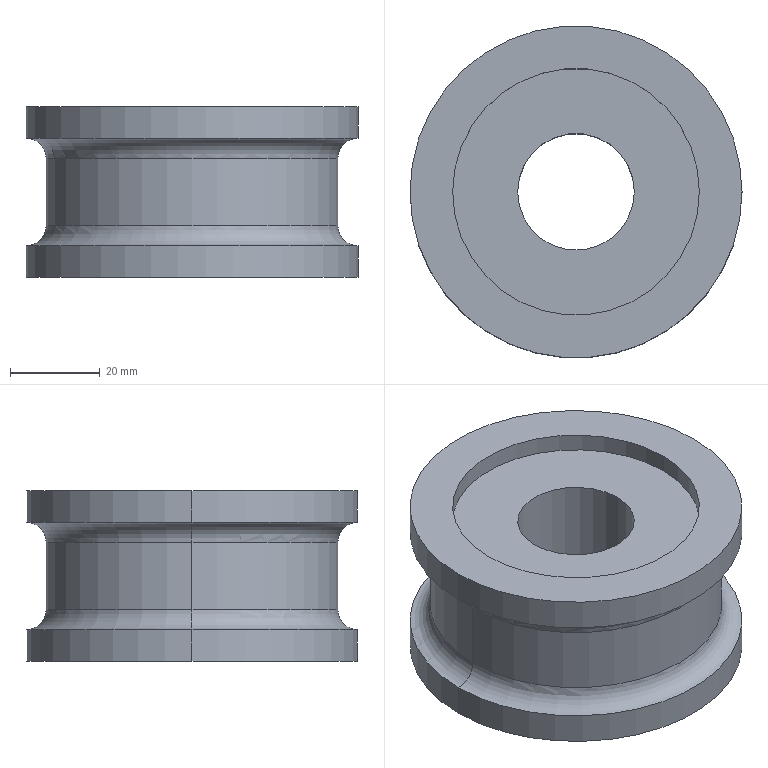Component | SolidWorks | 12AFlatGrooveSmallWheel-MillingAxis-1_12AFlatSlotSmallStraighteningWheel-1 | 1 solid | 20 faces | box 74 x 74 x 38 mm | volume 106746 mm3 | cylinder 12 | torus 4 | plane 4 | commonest cylinder face diameters 55 x4 74 x4 26 x2 65 x2 | material GCr15
build123d program:
from build123d import *


with BuildPart() as part:
    # Sketch1 → Revolve1 (revolve)
    with BuildSketch(Plane.XY, mode=Mode.PRIVATE) as revolve1_sk:
        with BuildLine():
            Line((0, 27.5), (0, 37))
            Line((0, 37), (7, 37))
            ThreePointArc((7, 37), (8.318, 33.818), (11.5, 32.5))
            Line((11.5, 32.5), (26.5, 32.5))
            ThreePointArc((26.5, 32.5), (29.682, 33.818), (31, 37))
            Line((31, 37), (38, 37))
            Line((38, 37), (38, 27.5))
            Line((38, 27.5), (34, 27.5))
            Line((34, 27.5), (34, 13))
            Line((34, 13), (4, 13))
            Line((4, 13), (4, 27.5))
            Line((4, 27.5), (0, 27.5))
        make_face()
    revolve(revolve1_sk.sketch.rotate(Axis((0, 0, 0), (1, 0, 0)), 90), axis=Axis((0, 0, 0), (1, 0, 0)))


solid = part.part

# Placed as in the assembly
solid = solid.moved(Location((-170.402, 66.538, 55.75), (0, 90, 0)))
STEP:
#1=CARTESIAN_POINT('',(-7.221,2.62,0.8563));
#2=VERTEX_POINT('',#1);
#3=CARTESIAN_POINT('',(-6.197,2.62,0.8563));
#4=VERTEX_POINT('',#3);
#5=CARTESIAN_POINT('',(-6.709,2.62,0.8563));
#6=DIRECTION('',(0.,0.,1.));
#7=DIRECTION('',(1.,0.,0.));
#8=AXIS2_PLACEMENT_3D('',#5,#6,#7);
#9=CIRCLE('',#8,0.5118);
#10=EDGE_CURVE('',#2,#4,#9,.T.);
#11=ORIENTED_EDGE('',*,*,#10,.F.);
#12=CARTESIAN_POINT('',(-7.221,2.62,2.037));
#13=VERTEX_POINT('',#12);
#14=CARTESIAN_POINT('',(-7.221,2.62,2.195));
#15=DIRECTION('',(0.,0.,1.));
#16=VECTOR('',#15,39.37);
#17=LINE('',#14,#16);
#18=EDGE_CURVE('',#2,#13,#17,.T.);
#19=ORIENTED_EDGE('',*,*,#18,.T.);
#20=CARTESIAN_POINT('',(-6.197,2.62,2.037));
#21=VERTEX_POINT('',#20);
#22=CARTESIAN_POINT('',(-6.709,2.62,2.037));
#23=DIRECTION('',(0.,0.,1.));
#24=DIRECTION('',(1.,0.,0.));
#25=AXIS2_PLACEMENT_3D('',#22,#23,#24);
#26=CIRCLE('',#25,0.5118);
#27=EDGE_CURVE('',#13,#21,#26,.T.);
#28=ORIENTED_EDGE('',*,*,#27,.T.);
#29=CARTESIAN_POINT('',(-6.197,2.62,2.195));
#30=DIRECTION('',(0.,0.,1.));
#31=VECTOR('',#30,39.37);
#32=LINE('',#29,#31);
#33=EDGE_CURVE('',#4,#21,#32,.T.);
#34=ORIENTED_EDGE('',*,*,#33,.F.);
#35=EDGE_LOOP('',(#11,#19,#28,#34));
#36=FACE_OUTER_BOUND('',#35,.T.);
#37=CARTESIAN_POINT('',(-6.709,2.62,2.195));
#38=DIRECTION('',(0.,0.,1.));
#39=DIRECTION('',(1.,0.,0.));
#40=AXIS2_PLACEMENT_3D('',#37,#38,#39);
#41=CYLINDRICAL_SURFACE('',#40,0.5118);
#42=ADVANCED_FACE('',(#36),#41,.F.);
#43=CARTESIAN_POINT('',(-7.791,2.62,2.037));
#44=VERTEX_POINT('',#43);
#45=CARTESIAN_POINT('',(-5.626,2.62,2.037));
#46=VERTEX_POINT('',#45);
#47=CARTESIAN_POINT('',(-6.709,2.62,2.037));
#48=DIRECTION('',(0.,0.,1.));
#49=DIRECTION('',(1.,0.,0.));
#50=AXIS2_PLACEMENT_3D('',#47,#48,#49);
#51=CIRCLE('',#50,1.083);
#52=EDGE_CURVE('',#44,#46,#51,.T.);
#53=ORIENTED_EDGE('',*,*,#52,.F.);
#54=CARTESIAN_POINT('',(-7.791,2.62,2.195));
#55=VERTEX_POINT('',#54);
#56=CARTESIAN_POINT('',(-7.791,2.62,2.195));
#57=DIRECTION('',(0.,0.,1.));
#58=VECTOR('',#57,39.37);
#59=LINE('',#56,#58);
#60=EDGE_CURVE('',#44,#55,#59,.T.);
#61=ORIENTED_EDGE('',*,*,#60,.T.);
#62=CARTESIAN_POINT('',(-5.626,2.62,2.195));
#63=VERTEX_POINT('',#62);
#64=CARTESIAN_POINT('',(-6.709,2.62,2.195));
#65=DIRECTION('',(0.,0.,1.));
#66=DIRECTION('',(1.,0.,0.));
#67=AXIS2_PLACEMENT_3D('',#64,#65,#66);
#68=CIRCLE('',#67,1.083);
#69=EDGE_CURVE('',#55,#63,#68,.T.);
#70=ORIENTED_EDGE('',*,*,#69,.T.);
#71=CARTESIAN_POINT('',(-5.626,2.62,2.195));
#72=DIRECTION('',(0.,0.,1.));
#73=VECTOR('',#72,39.37);
#74=LINE('',#71,#73);
#75=EDGE_CURVE('',#46,#63,#74,.T.);
#76=ORIENTED_EDGE('',*,*,#75,.F.);
#77=EDGE_LOOP('',(#53,#61,#70,#76));
#78=FACE_OUTER_BOUND('',#77,.T.);
#79=CARTESIAN_POINT('',(-6.709,2.62,2.195));
#80=DIRECTION('',(0.,0.,1.));
#81=DIRECTION('',(1.,0.,0.));
#82=AXIS2_PLACEMENT_3D('',#79,#80,#81);
#83=CYLINDRICAL_SURFACE('',#82,1.083);
#84=ADVANCED_FACE('',(#78),#83,.F.);
#85=CARTESIAN_POINT('',(-5.252,2.62,1.919));
#86=VERTEX_POINT('',#85);
#87=CARTESIAN_POINT('',(-8.165,2.62,1.919));
#88=VERTEX_POINT('',#87);
#89=CARTESIAN_POINT('',(-6.709,2.62,1.919));
#90=DIRECTION('',(0.,0.,1.));
#91=DIRECTION('',(1.,0.,0.));
#92=AXIS2_PLACEMENT_3D('',#89,#90,#91);
#93=CIRCLE('',#92,1.457);
#94=EDGE_CURVE('',#86,#88,#93,.T.);
#95=ORIENTED_EDGE('',*,*,#94,.T.);
#96=CARTESIAN_POINT('',(-8.165,2.62,2.195));
#97=VERTEX_POINT('',#96);
#98=CARTESIAN_POINT('',(-8.165,2.62,2.195));
#99=DIRECTION('',(0.,0.,1.));
#100=VECTOR('',#99,39.37);
#101=LINE('',#98,#100);
#102=EDGE_CURVE('',#88,#97,#101,.T.);
#103=ORIENTED_EDGE('',*,*,#102,.T.);
#104=CARTESIAN_POINT('',(-5.252,2.62,2.195));
#105=VERTEX_POINT('',#104);
#106=CARTESIAN_POINT('',(-6.709,2.62,2.195));
#107=DIRECTION('',(0.,0.,1.));
#108=DIRECTION('',(1.,0.,0.));
#109=AXIS2_PLACEMENT_3D('',#106,#107,#108);
#110=CIRCLE('',#109,1.457);
#111=EDGE_CURVE('',#105,#97,#110,.T.);
#112=ORIENTED_EDGE('',*,*,#111,.F.);
#113=CARTESIAN_POINT('',(-5.252,2.62,2.195));
#114=DIRECTION('',(0.,0.,1.));
#115=VECTOR('',#114,39.37);
#116=LINE('',#113,#115);
#117=EDGE_CURVE('',#86,#105,#116,.T.);
#118=ORIENTED_EDGE('',*,*,#117,.F.);
#119=EDGE_LOOP('',(#95,#103,#112,#118));
#120=FACE_OUTER_BOUND('',#119,.T.);
#121=CARTESIAN_POINT('',(-6.709,2.62,2.195));
#122=DIRECTION('',(0.,0.,1.));
#123=DIRECTION('',(1.,0.,0.));
#124=AXIS2_PLACEMENT_3D('',#121,#122,#123);
#125=CYLINDRICAL_SURFACE('',#124,1.457);
#126=ADVANCED_FACE('',(#120),#125,.T.);
#127=CARTESIAN_POINT('',(-6.709,2.62,1.919));
#128=DIRECTION('',(0.,0.,1.));
#129=DIRECTION('',(1.,0.,0.));
#130=AXIS2_PLACEMENT_3D('',#127,#128,#129);
#131=CIRCLE('',#130,1.457);
#132=EDGE_CURVE('',#88,#86,#131,.T.);
#133=ORIENTED_EDGE('',*,*,#132,.F.);
#134=CARTESIAN_POINT('',(-7.988,2.62,1.742));
#135=VERTEX_POINT('',#134);
#136=CARTESIAN_POINT('',(-8.165,2.62,1.742));
#137=DIRECTION('',(0.,1.,0.));
#138=DIRECTION('',(-1.,0.,0.));
#139=AXIS2_PLACEMENT_3D('',#136,#137,#138);
#140=CIRCLE('',#139,0.1772);
#141=EDGE_CURVE('',#88,#135,#140,.T.);
#142=ORIENTED_EDGE('',*,*,#141,.T.);
#143=CARTESIAN_POINT('',(-5.429,2.62,1.742));
#144=VERTEX_POINT('',#143);
#145=CARTESIAN_POINT('',(-6.709,2.62,1.742));
#146=DIRECTION('',(0.,0.,1.));
#147=DIRECTION('',(1.,0.,0.));
#148=AXIS2_PLACEMENT_3D('',#145,#146,#147);
#149=CIRCLE('',#148,1.28);
#150=EDGE_CURVE('',#135,#144,#149,.T.);
#151=ORIENTED_EDGE('',*,*,#150,.T.);
#152=CARTESIAN_POINT('',(-5.252,2.62,1.742));
#153=DIRECTION('',(0.,-1.,0.));
#154=DIRECTION('',(0.,0.,-1.));
#155=AXIS2_PLACEMENT_3D('',#152,#153,#154);
#156=CIRCLE('',#155,0.1772);
#157=EDGE_CURVE('',#86,#144,#156,.T.);
#158=ORIENTED_EDGE('',*,*,#157,.F.);
#159=EDGE_LOOP('',(#133,#142,#151,#158));
#160=FACE_OUTER_BOUND('',#159,.T.);
#161=CARTESIAN_POINT('',(-6.709,2.62,1.742));
#162=DIRECTION('',(0.,0.,1.));
#163=DIRECTION('',(1.,0.,0.));
#164=AXIS2_PLACEMENT_3D('',#161,#162,#163);
#165=TOROIDAL_SURFACE('',#164,1.457,0.1772);
#166=ADVANCED_FACE('',(#160),#165,.F.);
#167=CARTESIAN_POINT('',(-5.429,2.62,1.152));
#168=VERTEX_POINT('',#167);
#169=CARTESIAN_POINT('',(-7.988,2.62,1.152));
#170=VERTEX_POINT('',#169);
#171=CARTESIAN_POINT('',(-6.709,2.62,1.152));
#172=DIRECTION('',(0.,0.,1.));
#173=DIRECTION('',(1.,0.,0.));
#174=AXIS2_PLACEMENT_3D('',#171,#172,#173);
#175=CIRCLE('',#174,1.28);
#176=EDGE_CURVE('',#168,#170,#175,.T.);
#177=ORIENTED_EDGE('',*,*,#176,.T.);
#178=CARTESIAN_POINT('',(-7.988,2.62,2.195));
#179=DIRECTION('',(0.,0.,1.));
#180=VECTOR('',#179,39.37);
#181=LINE('',#178,#180);
#182=EDGE_CURVE('',#170,#135,#181,.T.);
#183=ORIENTED_EDGE('',*,*,#182,.T.);
#184=CARTESIAN_POINT('',(-6.709,2.62,1.742));
#185=DIRECTION('',(0.,0.,1.));
#186=DIRECTION('',(1.,0.,0.));
#187=AXIS2_PLACEMENT_3D('',#184,#185,#186);
#188=CIRCLE('',#187,1.28);
#189=EDGE_CURVE('',#144,#135,#188,.T.);
#190=ORIENTED_EDGE('',*,*,#189,.F.);
#191=CARTESIAN_POINT('',(-5.429,2.62,2.195));
#192=DIRECTION('',(0.,0.,1.));
#193=VECTOR('',#192,39.37);
#194=LINE('',#191,#193);
#195=EDGE_CURVE('',#168,#144,#194,.T.);
#196=ORIENTED_EDGE('',*,*,#195,.F.);
#197=EDGE_LOOP('',(#177,#183,#190,#196));
#198=FACE_OUTER_BOUND('',#197,.T.);
#199=CARTESIAN_POINT('',(-6.709,2.62,2.195));
#200=DIRECTION('',(0.,0.,1.));
#201=DIRECTION('',(1.,0.,0.));
#202=AXIS2_PLACEMENT_3D('',#199,#200,#201);
#203=CYLINDRICAL_SURFACE('',#202,1.28);
#204=ADVANCED_FACE('',(#198),#203,.T.);
#205=CARTESIAN_POINT('',(-6.709,2.62,1.152));
#206=DIRECTION('',(0.,0.,1.));
#207=DIRECTION('',(1.,0.,0.));
#208=AXIS2_PLACEMENT_3D('',#205,#206,#207);
#209=CIRCLE('',#208,1.28);
#210=EDGE_CURVE('',#170,#168,#209,.T.);
#211=ORIENTED_EDGE('',*,*,#210,.F.);
#212=CARTESIAN_POINT('',(-8.165,2.62,0.9744));
#213=VERTEX_POINT('',#212);
#214=CARTESIAN_POINT('',(-8.165,2.62,1.152));
#215=DIRECTION('',(0.,1.,0.));
#216=DIRECTION('',(-1.,0.,0.));
#217=AXIS2_PLACEMENT_3D('',#214,#215,#216);
#218=CIRCLE('',#217,0.1772);
#219=EDGE_CURVE('',#170,#213,#218,.T.);
#220=ORIENTED_EDGE('',*,*,#219,.T.);
#221=CARTESIAN_POINT('',(-5.252,2.62,0.9744));
#222=VERTEX_POINT('',#221);
#223=CARTESIAN_POINT('',(-6.709,2.62,0.9744));
#224=DIRECTION('',(0.,0.,1.));
#225=DIRECTION('',(1.,0.,0.));
#226=AXIS2_PLACEMENT_3D('',#223,#224,#225);
#227=CIRCLE('',#226,1.457);
#228=EDGE_CURVE('',#213,#222,#227,.T.);
#229=ORIENTED_EDGE('',*,*,#228,.T.);
#230=CARTESIAN_POINT('',(-5.252,2.62,1.152));
#231=DIRECTION('',(0.,-1.,0.));
#232=DIRECTION('',(0.,0.,-1.));
#233=AXIS2_PLACEMENT_3D('',#230,#231,#232);
#234=CIRCLE('',#233,0.1772);
#235=EDGE_CURVE('',#168,#222,#234,.T.);
#236=ORIENTED_EDGE('',*,*,#235,.F.);
#237=EDGE_LOOP('',(#211,#220,#229,#236));
#238=FACE_OUTER_BOUND('',#237,.T.);
#239=CARTESIAN_POINT('',(-6.709,2.62,1.152));
#240=DIRECTION('',(0.,0.,1.));
#241=DIRECTION('',(1.,0.,0.));
#242=AXIS2_PLACEMENT_3D('',#239,#240,#241);
#243=TOROIDAL_SURFACE('',#242,1.457,0.1772);
#244=ADVANCED_FACE('',(#238),#243,.F.);
#245=CARTESIAN_POINT('',(-5.252,2.62,0.6988));
#246=VERTEX_POINT('',#245);
#247=CARTESIAN_POINT('',(-8.165,2.62,0.6988));
#248=VERTEX_POINT('',#247);
#249=CARTESIAN_POINT('',(-6.709,2.62,0.6988));
#250=DIRECTION('',(0.,0.,1.));
#251=DIRECTION('',(1.,0.,0.));
#252=AXIS2_PLACEMENT_3D('',#249,#250,#251);
#253=CIRCLE('',#252,1.457);
#254=EDGE_CURVE('',#246,#248,#253,.T.);
#255=ORIENTED_EDGE('',*,*,#254,.T.);
#256=CARTESIAN_POINT('',(-8.165,2.62,2.195));
#257=DIRECTION('',(0.,0.,1.));
#258=VECTOR('',#257,39.37);
#259=LINE('',#256,#258);
#260=EDGE_CURVE('',#248,#213,#259,.T.);
#261=ORIENTED_EDGE('',*,*,#260,.T.);
#262=CARTESIAN_POINT('',(-6.709,2.62,0.9744));
#263=DIRECTION('',(0.,0.,1.));
#264=DIRECTION('',(1.,0.,0.));
#265=AXIS2_PLACEMENT_3D('',#262,#263,#264);
#266=CIRCLE('',#265,1.457);
#267=EDGE_CURVE('',#222,#213,#266,.T.);
#268=ORIENTED_EDGE('',*,*,#267,.F.);
#269=CARTESIAN_POINT('',(-5.252,2.62,2.195));
#270=DIRECTION('',(0.,0.,1.));
#271=VECTOR('',#270,39.37);
#272=LINE('',#269,#271);
#273=EDGE_CURVE('',#246,#222,#272,.T.);
#274=ORIENTED_EDGE('',*,*,#273,.F.);
#275=EDGE_LOOP('',(#255,#261,#268,#274));
#276=FACE_OUTER_BOUND('',#275,.T.);
#277=CARTESIAN_POINT('',(-6.709,2.62,2.195));
#278=DIRECTION('',(0.,0.,1.));
#279=DIRECTION('',(1.,0.,0.));
#280=AXIS2_PLACEMENT_3D('',#277,#278,#279);
#281=CYLINDRICAL_SURFACE('',#280,1.457);
#282=ADVANCED_FACE('',(#276),#281,.T.);
#283=CARTESIAN_POINT('',(-7.791,2.62,0.6988));
#284=VERTEX_POINT('',#283);
#285=CARTESIAN_POINT('',(-5.626,2.62,0.6988));
#286=VERTEX_POINT('',#285);
#287=CARTESIAN_POINT('',(-6.709,2.62,0.6988));
#288=DIRECTION('',(0.,0.,1.));
#289=DIRECTION('',(1.,0.,0.));
#290=AXIS2_PLACEMENT_3D('',#287,#288,#289);
#291=CIRCLE('',#290,1.083);
#292=EDGE_CURVE('',#284,#286,#291,.T.);
#293=ORIENTED_EDGE('',*,*,#292,.F.);
#294=CARTESIAN_POINT('',(-7.791,2.62,0.8563));
#295=VERTEX_POINT('',#294);
#296=CARTESIAN_POINT('',(-7.791,2.62,2.195));
#297=DIRECTION('',(0.,0.,1.));
#298=VECTOR('',#297,39.37);
#299=LINE('',#296,#298);
#300=EDGE_CURVE('',#284,#295,#299,.T.);
#301=ORIENTED_EDGE('',*,*,#300,.T.);
#302=CARTESIAN_POINT('',(-5.626,2.62,0.8563));
#303=VERTEX_POINT('',#302);
#304=CARTESIAN_POINT('',(-6.709,2.62,0.8563));
#305=DIRECTION('',(0.,0.,1.));
#306=DIRECTION('',(1.,0.,0.));
#307=AXIS2_PLACEMENT_3D('',#304,#305,#306);
#308=CIRCLE('',#307,1.083);
#309=EDGE_CURVE('',#295,#303,#308,.T.);
#310=ORIENTED_EDGE('',*,*,#309,.T.);
#311=CARTESIAN_POINT('',(-5.626,2.62,2.195));
#312=DIRECTION('',(0.,0.,1.));
#313=VECTOR('',#312,39.37);
#314=LINE('',#311,#313);
#315=EDGE_CURVE('',#286,#303,#314,.T.);
#316=ORIENTED_EDGE('',*,*,#315,.F.);
#317=EDGE_LOOP('',(#293,#301,#310,#316));
#318=FACE_OUTER_BOUND('',#317,.T.);
#319=CARTESIAN_POINT('',(-6.709,2.62,2.195));
#320=DIRECTION('',(0.,0.,1.));
#321=DIRECTION('',(1.,0.,0.));
#322=AXIS2_PLACEMENT_3D('',#319,#320,#321);
#323=CYLINDRICAL_SURFACE('',#322,1.083);
#324=ADVANCED_FACE('',(#318),#323,.F.);
#325=CARTESIAN_POINT('',(-6.709,2.62,0.8563));
#326=DIRECTION('',(0.,0.,1.));
#327=DIRECTION('',(1.,0.,0.));
#328=AXIS2_PLACEMENT_3D('',#325,#326,#327);
#329=CIRCLE('',#328,1.083);
#330=EDGE_CURVE('',#303,#295,#329,.T.);
#331=ORIENTED_EDGE('',*,*,#330,.F.);
#332=ORIENTED_EDGE('',*,*,#309,.F.);
#333=EDGE_LOOP('',(#331,#332));
#334=FACE_OUTER_BOUND('',#333,.T.);
#335=CARTESIAN_POINT('',(-6.709,2.62,0.8563));
#336=DIRECTION('',(0.,0.,1.));
#337=DIRECTION('',(1.,0.,0.));
#338=AXIS2_PLACEMENT_3D('',#335,#336,#337);
#339=CIRCLE('',#338,0.5118);
#340=EDGE_CURVE('',#4,#2,#339,.T.);
#341=ORIENTED_EDGE('',*,*,#340,.T.);
#342=ORIENTED_EDGE('',*,*,#10,.T.);
#343=EDGE_LOOP('',(#341,#342));
#344=FACE_BOUND('',#343,.T.);
#345=CARTESIAN_POINT('',(-6.709,3.131,0.8563));
#346=DIRECTION('',(0.,0.,1.));
#347=DIRECTION('',(1.,0.,0.));
#348=AXIS2_PLACEMENT_3D('',#345,#346,#347);
#349=PLANE('',#348);
#350=ADVANCED_FACE('',(#334,#344),#349,.F.);
#351=ORIENTED_EDGE('',*,*,#300,.F.);
#352=CARTESIAN_POINT('',(-6.709,2.62,0.6988));
#353=DIRECTION('',(0.,0.,1.));
#354=DIRECTION('',(1.,0.,0.));
#355=AXIS2_PLACEMENT_3D('',#352,#353,#354);
#356=CIRCLE('',#355,1.083);
#357=EDGE_CURVE('',#286,#284,#356,.T.);
#358=ORIENTED_EDGE('',*,*,#357,.F.);
#359=ORIENTED_EDGE('',*,*,#315,.T.);
#360=ORIENTED_EDGE('',*,*,#330,.T.);
#361=EDGE_LOOP('',(#351,#358,#359,#360));
#362=FACE_OUTER_BOUND('',#361,.T.);
#363=CARTESIAN_POINT('',(-6.709,2.62,2.195));
#364=DIRECTION('',(0.,0.,1.));
#365=DIRECTION('',(1.,0.,0.));
#366=AXIS2_PLACEMENT_3D('',#363,#364,#365);
#367=CYLINDRICAL_SURFACE('',#366,1.083);
#368=ADVANCED_FACE('',(#362),#367,.F.);
#369=ORIENTED_EDGE('',*,*,#254,.F.);
#370=CARTESIAN_POINT('',(-6.709,2.62,0.6988));
#371=DIRECTION('',(0.,0.,1.));
#372=DIRECTION('',(1.,0.,0.));
#373=AXIS2_PLACEMENT_3D('',#370,#371,#372);
#374=CIRCLE('',#373,1.457);
#375=EDGE_CURVE('',#248,#246,#374,.T.);
#376=ORIENTED_EDGE('',*,*,#375,.F.);
#377=EDGE_LOOP('',(#369,#376));
#378=FACE_OUTER_BOUND('',#377,.T.);
#379=ORIENTED_EDGE('',*,*,#357,.T.);
#380=ORIENTED_EDGE('',*,*,#292,.T.);
#381=EDGE_LOOP('',(#379,#380));
#382=FACE_BOUND('',#381,.T.);
#383=CARTESIAN_POINT('',(-6.709,4.076,0.6988));
#384=DIRECTION('',(0.,0.,1.));
#385=DIRECTION('',(1.,0.,0.));
#386=AXIS2_PLACEMENT_3D('',#383,#384,#385);
#387=PLANE('',#386);
#388=ADVANCED_FACE('',(#378,#382),#387,.F.);
#389=ORIENTED_EDGE('',*,*,#260,.F.);
#390=ORIENTED_EDGE('',*,*,#375,.T.);
#391=ORIENTED_EDGE('',*,*,#273,.T.);
#392=ORIENTED_EDGE('',*,*,#228,.F.);
#393=EDGE_LOOP('',(#389,#390,#391,#392));
#394=FACE_OUTER_BOUND('',#393,.T.);
#395=CARTESIAN_POINT('',(-6.709,2.62,2.195));
#396=DIRECTION('',(0.,0.,1.));
#397=DIRECTION('',(1.,0.,0.));
#398=AXIS2_PLACEMENT_3D('',#395,#396,#397);
#399=CYLINDRICAL_SURFACE('',#398,1.457);
#400=ADVANCED_FACE('',(#394),#399,.T.);
#401=ORIENTED_EDGE('',*,*,#219,.F.);
#402=ORIENTED_EDGE('',*,*,#176,.F.);
#403=ORIENTED_EDGE('',*,*,#235,.T.);
#404=ORIENTED_EDGE('',*,*,#267,.T.);
#405=EDGE_LOOP('',(#401,#402,#403,#404));
#406=FACE_OUTER_BOUND('',#405,.T.);
#407=CARTESIAN_POINT('',(-6.709,2.62,1.152));
#408=DIRECTION('',(0.,0.,1.));
#409=DIRECTION('',(1.,0.,0.));
#410=AXIS2_PLACEMENT_3D('',#407,#408,#409);
#411=TOROIDAL_SURFACE('',#410,1.457,0.1772);
#412=ADVANCED_FACE('',(#406),#411,.F.);
#413=ORIENTED_EDGE('',*,*,#182,.F.);
#414=ORIENTED_EDGE('',*,*,#210,.T.);
#415=ORIENTED_EDGE('',*,*,#195,.T.);
#416=ORIENTED_EDGE('',*,*,#150,.F.);
#417=EDGE_LOOP('',(#413,#414,#415,#416));
#418=FACE_OUTER_BOUND('',#417,.T.);
#419=CARTESIAN_POINT('',(-6.709,2.62,2.195));
#420=DIRECTION('',(0.,0.,1.));
#421=DIRECTION('',(1.,0.,0.));
#422=AXIS2_PLACEMENT_3D('',#419,#420,#421);
#423=CYLINDRICAL_SURFACE('',#422,1.28);
#424=ADVANCED_FACE('',(#418),#423,.T.);
#425=ORIENTED_EDGE('',*,*,#141,.F.);
#426=ORIENTED_EDGE('',*,*,#94,.F.);
#427=ORIENTED_EDGE('',*,*,#157,.T.);
#428=ORIENTED_EDGE('',*,*,#189,.T.);
#429=EDGE_LOOP('',(#425,#426,#427,#428));
#430=FACE_OUTER_BOUND('',#429,.T.);
#431=CARTESIAN_POINT('',(-6.709,2.62,1.742));
#432=DIRECTION('',(0.,0.,1.));
#433=DIRECTION('',(1.,0.,0.));
#434=AXIS2_PLACEMENT_3D('',#431,#432,#433);
#435=TOROIDAL_SURFACE('',#434,1.457,0.1772);
#436=ADVANCED_FACE('',(#430),#435,.F.);
#437=ORIENTED_EDGE('',*,*,#102,.F.);
#438=ORIENTED_EDGE('',*,*,#132,.T.);
#439=ORIENTED_EDGE('',*,*,#117,.T.);
#440=CARTESIAN_POINT('',(-6.709,2.62,2.195));
#441=DIRECTION('',(0.,0.,1.));
#442=DIRECTION('',(1.,0.,0.));
#443=AXIS2_PLACEMENT_3D('',#440,#441,#442);
#444=CIRCLE('',#443,1.457);
#445=EDGE_CURVE('',#97,#105,#444,.T.);
#446=ORIENTED_EDGE('',*,*,#445,.F.);
#447=EDGE_LOOP('',(#437,#438,#439,#446));
#448=FACE_OUTER_BOUND('',#447,.T.);
#449=CARTESIAN_POINT('',(-6.709,2.62,2.195));
#450=DIRECTION('',(0.,0.,1.));
#451=DIRECTION('',(1.,0.,0.));
#452=AXIS2_PLACEMENT_3D('',#449,#450,#451);
#453=CYLINDRICAL_SURFACE('',#452,1.457);
#454=ADVANCED_FACE('',(#448),#453,.T.);
#455=CARTESIAN_POINT('',(-6.709,2.62,2.195));
#456=DIRECTION('',(0.,0.,1.));
#457=DIRECTION('',(1.,0.,0.));
#458=AXIS2_PLACEMENT_3D('',#455,#456,#457);
#459=CIRCLE('',#458,1.083);
#460=EDGE_CURVE('',#63,#55,#459,.T.);
#461=ORIENTED_EDGE('',*,*,#460,.F.);
#462=ORIENTED_EDGE('',*,*,#69,.F.);
#463=EDGE_LOOP('',(#461,#462));
#464=FACE_BOUND('',#463,.T.);
#465=ORIENTED_EDGE('',*,*,#111,.T.);
#466=ORIENTED_EDGE('',*,*,#445,.T.);
#467=EDGE_LOOP('',(#465,#466));
#468=FACE_OUTER_BOUND('',#467,.T.);
#469=CARTESIAN_POINT('',(-6.709,3.702,2.195));
#470=DIRECTION('',(0.,0.,-1.));
#471=DIRECTION('',(-1.,0.,0.));
#472=AXIS2_PLACEMENT_3D('',#469,#470,#471);
#473=PLANE('',#472);
#474=ADVANCED_FACE('',(#464,#468),#473,.F.);
#475=ORIENTED_EDGE('',*,*,#60,.F.);
#476=CARTESIAN_POINT('',(-6.709,2.62,2.037));
#477=DIRECTION('',(0.,0.,1.));
#478=DIRECTION('',(1.,0.,0.));
#479=AXIS2_PLACEMENT_3D('',#476,#477,#478);
#480=CIRCLE('',#479,1.083);
#481=EDGE_CURVE('',#46,#44,#480,.T.);
#482=ORIENTED_EDGE('',*,*,#481,.F.);
#483=ORIENTED_EDGE('',*,*,#75,.T.);
#484=ORIENTED_EDGE('',*,*,#460,.T.);
#485=EDGE_LOOP('',(#475,#482,#483,#484));
#486=FACE_OUTER_BOUND('',#485,.T.);
#487=CARTESIAN_POINT('',(-6.709,2.62,2.195));
#488=DIRECTION('',(0.,0.,1.));
#489=DIRECTION('',(1.,0.,0.));
#490=AXIS2_PLACEMENT_3D('',#487,#488,#489);
#491=CYLINDRICAL_SURFACE('',#490,1.083);
#492=ADVANCED_FACE('',(#486),#491,.F.);
#493=CARTESIAN_POINT('',(-6.709,2.62,2.037));
#494=DIRECTION('',(0.,0.,1.));
#495=DIRECTION('',(1.,0.,0.));
#496=AXIS2_PLACEMENT_3D('',#493,#494,#495);
#497=CIRCLE('',#496,0.5118);
#498=EDGE_CURVE('',#21,#13,#497,.T.);
#499=ORIENTED_EDGE('',*,*,#498,.F.);
#500=ORIENTED_EDGE('',*,*,#27,.F.);
#501=EDGE_LOOP('',(#499,#500));
#502=FACE_BOUND('',#501,.T.);
#503=ORIENTED_EDGE('',*,*,#481,.T.);
#504=ORIENTED_EDGE('',*,*,#52,.T.);
#505=EDGE_LOOP('',(#503,#504));
#506=FACE_OUTER_BOUND('',#505,.T.);
#507=CARTESIAN_POINT('',(-6.709,3.702,2.037));
#508=DIRECTION('',(0.,0.,-1.));
#509=DIRECTION('',(-1.,0.,0.));
#510=AXIS2_PLACEMENT_3D('',#507,#508,#509);
#511=PLANE('',#510);
#512=ADVANCED_FACE('',(#502,#506),#511,.F.);
#513=ORIENTED_EDGE('',*,*,#18,.F.);
#514=ORIENTED_EDGE('',*,*,#340,.F.);
#515=ORIENTED_EDGE('',*,*,#33,.T.);
#516=ORIENTED_EDGE('',*,*,#498,.T.);
#517=EDGE_LOOP('',(#513,#514,#515,#516));
#518=FACE_OUTER_BOUND('',#517,.T.);
#519=CARTESIAN_POINT('',(-6.709,2.62,2.195));
#520=DIRECTION('',(0.,0.,1.));
#521=DIRECTION('',(1.,0.,0.));
#522=AXIS2_PLACEMENT_3D('',#519,#520,#521);
#523=CYLINDRICAL_SURFACE('',#522,0.5118);
#524=ADVANCED_FACE('',(#518),#523,.F.);
#525=CLOSED_SHELL('',(#42,#84,#126,#166,#204,#244,#282,#324,#350,#368,#388,#400,#412,#424,#436,#454,#474,#492,#512,#524));
#526=MANIFOLD_SOLID_BREP('',#525);
#527=CARTESIAN_POINT('',(0.,0.,0.));
#528=DIRECTION('',(0.,0.,1.));
#529=DIRECTION('',(1.,0.,0.));
#530=AXIS2_PLACEMENT_3D('',#527,#528,#529);
#531=(LENGTH_UNIT()NAMED_UNIT(*)SI_UNIT($,.METRE.));
#532=LENGTH_MEASURE_WITH_UNIT(LENGTH_MEASURE(0.0254),#531);
#533=DIMENSIONAL_EXPONENTS(1.,0.,0.,0.,0.,0.,0.);
#534=(CONVERSION_BASED_UNIT('',#532)LENGTH_UNIT()NAMED_UNIT(#533));
#535=UNCERTAINTY_MEASURE_WITH_UNIT(LENGTH_MEASURE(0.00001),#534,'','');
#536=(NAMED_UNIT(*)PLANE_ANGLE_UNIT()SI_UNIT($,.RADIAN.));
#537=(NAMED_UNIT(*)SI_UNIT($,.STERADIAN.)SOLID_ANGLE_UNIT());
#538=(GEOMETRIC_REPRESENTATION_CONTEXT(3)GLOBAL_UNCERTAINTY_ASSIGNED_CONTEXT((#535))GLOBAL_UNIT_ASSIGNED_CONTEXT((#534,#536,#537))REPRESENTATION_CONTEXT('',''));
#539=ADVANCED_BREP_SHAPE_REPRESENTATION('',(#526,#530),#538);
#540=COLOUR_RGB('',0.7922,0.8196,0.9333);
#541=FILL_AREA_STYLE_COLOUR('',#540);
#542=FILL_AREA_STYLE('',(#541));
#543=SURFACE_STYLE_FILL_AREA(#542);
#544=SURFACE_SIDE_STYLE('',(#543));
#545=SURFACE_STYLE_USAGE(.BOTH.,#544);
#546=PRESENTATION_STYLE_ASSIGNMENT((#545));
#547=STYLED_ITEM('',(#546),#526);
#548=(LENGTH_UNIT()NAMED_UNIT(*)SI_UNIT($,.METRE.));
#549=LENGTH_MEASURE_WITH_UNIT(LENGTH_MEASURE(0.0254),#548);
#550=DIMENSIONAL_EXPONENTS(1.,0.,0.,0.,0.,0.,0.);
#551=(CONVERSION_BASED_UNIT('',#549)LENGTH_UNIT()NAMED_UNIT(#550));
#552=UNCERTAINTY_MEASURE_WITH_UNIT(LENGTH_MEASURE(0.00001),#551,'','');
#553=(NAMED_UNIT(*)PLANE_ANGLE_UNIT()SI_UNIT($,.RADIAN.));
#554=(NAMED_UNIT(*)SI_UNIT($,.STERADIAN.)SOLID_ANGLE_UNIT());
#555=(GEOMETRIC_REPRESENTATION_CONTEXT(3)GLOBAL_UNCERTAINTY_ASSIGNED_CONTEXT((#552))GLOBAL_UNIT_ASSIGNED_CONTEXT((#551,#553,#554))REPRESENTATION_CONTEXT('',''));
#556=MECHANICAL_DESIGN_GEOMETRIC_PRESENTATION_REPRESENTATION('',(#547),#555);
#557=PRESENTATION_LAYER_ASSIGNMENT('','',(#547));